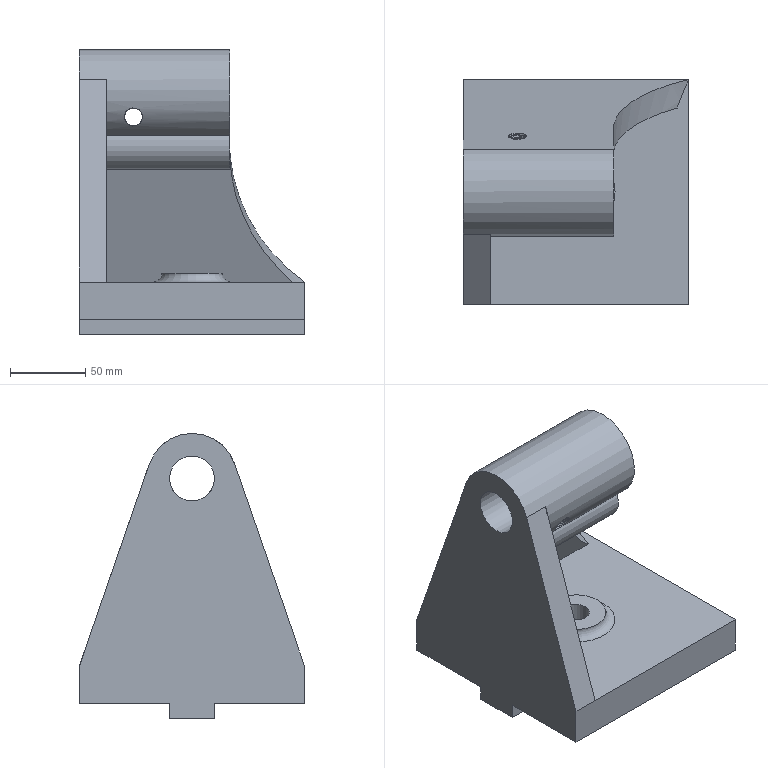Component | NX | BODY_1 | 1 solid | 181 faces | volume 1276162 mm3 | cylinder 108 | spline 49 | plane 23 | torus 1 | commonest cylinder face diameters 15 x55 12.1 x24 12 x22 30 x2 18 x1 4 x1 60 x1 250 x1